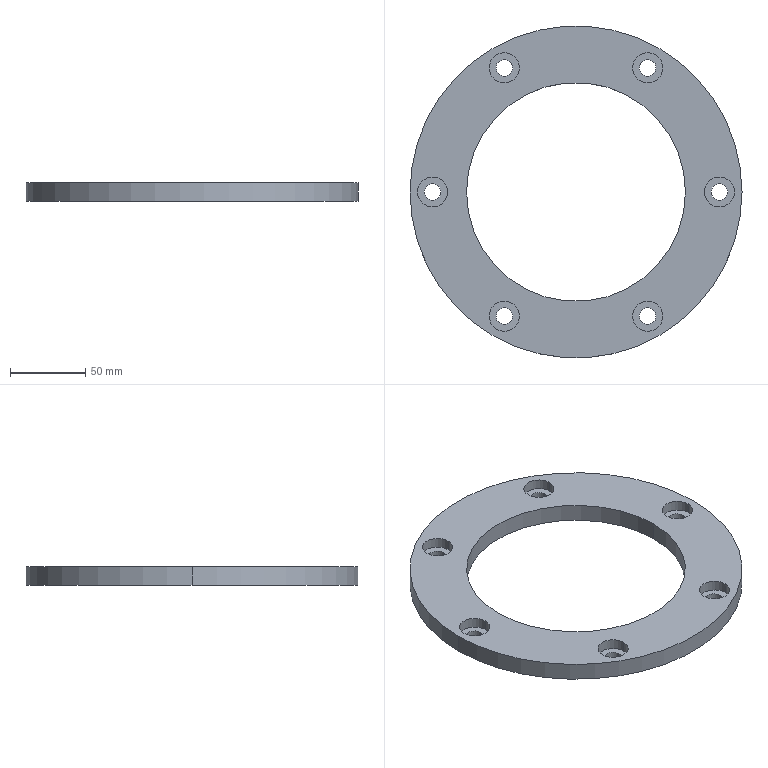Component | SolidWorks | PunchRetainer-1 | 1 solid | 36 faces | box 220 x 220 x 12 mm | volume 241958 mm3 | cylinder 28 | plane 8 | commonest cylinder face diameters 20 x12 11 x12 145 x2 220 x2
build123d program:
from build123d import *

# Parameters (mm, degrees)
SKETCH1_R           = 110
SKETCH1_R_2         = 72.5
SKETCH1_R_3         = 5.5
BOSS_EXTRUDE1_DEPTH = 12
SKETCH2_R           = 10
CUT_EXTRUDE1_DEPTH  = 7


with BuildPart() as part:
    # Sketch1 → Boss-Extrude1 (new body)
    with BuildSketch(Plane.XY):
        Circle(SKETCH1_R)
        Circle(SKETCH1_R_2, mode=Mode.SUBTRACT)
        with Locations((-95, 0)):
            Circle(SKETCH1_R_3, mode=Mode.SUBTRACT)
        with Locations((-47.5, 82.272)):
            Circle(SKETCH1_R_3, mode=Mode.SUBTRACT)
        with Locations((47.5, 82.272)):
            Circle(SKETCH1_R_3, mode=Mode.SUBTRACT)
        with Locations((95, 0)):
            Circle(SKETCH1_R_3, mode=Mode.SUBTRACT)
        with Locations((47.5, -82.272)):
            Circle(SKETCH1_R_3, mode=Mode.SUBTRACT)
        with Locations((-47.5, -82.272)):
            Circle(SKETCH1_R_3, mode=Mode.SUBTRACT)
    extrude(amount=BOSS_EXTRUDE1_DEPTH)

    # Sketch2 → Cut-Extrude1 (cut)
    with BuildSketch(Plane.XY.offset(12)):
        with Locations((-95, 0)):
            Circle(SKETCH2_R)
        with Locations((-47.5, 82.272)):
            Circle(SKETCH2_R)
        with Locations((47.5, 82.272)):
            Circle(SKETCH2_R)
        with Locations((95, 0)):
            Circle(SKETCH2_R)
        with Locations((47.5, -82.272)):
            Circle(SKETCH2_R)
        with Locations((-47.5, -82.272)):
            Circle(SKETCH2_R)
    extrude(amount=-CUT_EXTRUDE1_DEPTH, mode=Mode.SUBTRACT)


solid = part.part

# Placed as in the assembly
solid = solid.moved(Location((0, 0, -231), (0, 0, 0)))
STEP:
#1=COLOUR_RGB('',0.7922,0.8196,0.9333);
#2=FILL_AREA_STYLE_COLOUR('',#1);
#3=FILL_AREA_STYLE('',(#2));
#4=SURFACE_STYLE_FILL_AREA(#3);
#5=SURFACE_SIDE_STYLE('',(#4));
#6=SURFACE_STYLE_USAGE(.BOTH.,#5);
#7=PRESENTATION_STYLE_ASSIGNMENT((#6));
#8=CARTESIAN_POINT('',(-4.134,-0.,-8.898));
#9=VERTEX_POINT('',#8);
#10=CARTESIAN_POINT('',(-3.346,-0.,-8.898));
#11=VERTEX_POINT('',#10);
#12=CARTESIAN_POINT('',(-3.74,-0.,-8.898));
#13=DIRECTION('',(0.,0.,1.));
#14=DIRECTION('',(1.,0.,0.));
#15=AXIS2_PLACEMENT_3D('',#12,#13,#14);
#16=CIRCLE('',#15,0.3937);
#17=EDGE_CURVE('',#9,#11,#16,.T.);
#18=ORIENTED_EDGE('',*,*,#17,.F.);
#19=CARTESIAN_POINT('',(-4.134,-0.,-8.622));
#20=VERTEX_POINT('',#19);
#21=CARTESIAN_POINT('',(-4.134,-0.,-8.898));
#22=DIRECTION('',(0.,0.,1.));
#23=VECTOR('',#22,39.37);
#24=LINE('',#21,#23);
#25=EDGE_CURVE('',#9,#20,#24,.T.);
#26=ORIENTED_EDGE('',*,*,#25,.T.);
#27=CARTESIAN_POINT('',(-3.346,-0.,-8.622));
#28=VERTEX_POINT('',#27);
#29=CARTESIAN_POINT('',(-3.74,-0.,-8.622));
#30=DIRECTION('',(0.,0.,1.));
#31=DIRECTION('',(1.,0.,0.));
#32=AXIS2_PLACEMENT_3D('',#29,#30,#31);
#33=CIRCLE('',#32,0.3937);
#34=EDGE_CURVE('',#20,#28,#33,.T.);
#35=ORIENTED_EDGE('',*,*,#34,.T.);
#36=CARTESIAN_POINT('',(-3.346,-0.,-8.898));
#37=DIRECTION('',(0.,0.,1.));
#38=VECTOR('',#37,39.37);
#39=LINE('',#36,#38);
#40=EDGE_CURVE('',#11,#28,#39,.T.);
#41=ORIENTED_EDGE('',*,*,#40,.F.);
#42=EDGE_LOOP('',(#18,#26,#35,#41));
#43=FACE_OUTER_BOUND('',#42,.T.);
#44=CARTESIAN_POINT('',(-3.74,-0.,-8.898));
#45=DIRECTION('',(0.,0.,1.));
#46=DIRECTION('',(1.,0.,0.));
#47=AXIS2_PLACEMENT_3D('',#44,#45,#46);
#48=CYLINDRICAL_SURFACE('',#47,0.3937);
#49=ADVANCED_FACE('',(#43),#48,.F.);
#50=CARTESIAN_POINT('',(-2.264,3.239,-8.898));
#51=VERTEX_POINT('',#50);
#52=CARTESIAN_POINT('',(-1.476,3.239,-8.898));
#53=VERTEX_POINT('',#52);
#54=CARTESIAN_POINT('',(-1.87,3.239,-8.898));
#55=DIRECTION('',(0.,0.,1.));
#56=DIRECTION('',(1.,0.,0.));
#57=AXIS2_PLACEMENT_3D('',#54,#55,#56);
#58=CIRCLE('',#57,0.3937);
#59=EDGE_CURVE('',#51,#53,#58,.T.);
#60=ORIENTED_EDGE('',*,*,#59,.F.);
#61=CARTESIAN_POINT('',(-2.264,3.239,-8.622));
#62=VERTEX_POINT('',#61);
#63=CARTESIAN_POINT('',(-2.264,3.239,-8.898));
#64=DIRECTION('',(0.,0.,1.));
#65=VECTOR('',#64,39.37);
#66=LINE('',#63,#65);
#67=EDGE_CURVE('',#51,#62,#66,.T.);
#68=ORIENTED_EDGE('',*,*,#67,.T.);
#69=CARTESIAN_POINT('',(-1.476,3.239,-8.622));
#70=VERTEX_POINT('',#69);
#71=CARTESIAN_POINT('',(-1.87,3.239,-8.622));
#72=DIRECTION('',(0.,0.,1.));
#73=DIRECTION('',(1.,0.,0.));
#74=AXIS2_PLACEMENT_3D('',#71,#72,#73);
#75=CIRCLE('',#74,0.3937);
#76=EDGE_CURVE('',#62,#70,#75,.T.);
#77=ORIENTED_EDGE('',*,*,#76,.T.);
#78=CARTESIAN_POINT('',(-1.476,3.239,-8.898));
#79=DIRECTION('',(0.,0.,1.));
#80=VECTOR('',#79,39.37);
#81=LINE('',#78,#80);
#82=EDGE_CURVE('',#53,#70,#81,.T.);
#83=ORIENTED_EDGE('',*,*,#82,.F.);
#84=EDGE_LOOP('',(#60,#68,#77,#83));
#85=FACE_OUTER_BOUND('',#84,.T.);
#86=CARTESIAN_POINT('',(-1.87,3.239,-8.898));
#87=DIRECTION('',(0.,0.,1.));
#88=DIRECTION('',(1.,0.,0.));
#89=AXIS2_PLACEMENT_3D('',#86,#87,#88);
#90=CYLINDRICAL_SURFACE('',#89,0.3937);
#91=ADVANCED_FACE('',(#85),#90,.F.);
#92=CARTESIAN_POINT('',(1.476,3.239,-8.898));
#93=VERTEX_POINT('',#92);
#94=CARTESIAN_POINT('',(2.264,3.239,-8.898));
#95=VERTEX_POINT('',#94);
#96=CARTESIAN_POINT('',(1.87,3.239,-8.898));
#97=DIRECTION('',(0.,0.,1.));
#98=DIRECTION('',(1.,0.,0.));
#99=AXIS2_PLACEMENT_3D('',#96,#97,#98);
#100=CIRCLE('',#99,0.3937);
#101=EDGE_CURVE('',#93,#95,#100,.T.);
#102=ORIENTED_EDGE('',*,*,#101,.F.);
#103=CARTESIAN_POINT('',(1.476,3.239,-8.622));
#104=VERTEX_POINT('',#103);
#105=CARTESIAN_POINT('',(1.476,3.239,-8.898));
#106=DIRECTION('',(0.,0.,1.));
#107=VECTOR('',#106,39.37);
#108=LINE('',#105,#107);
#109=EDGE_CURVE('',#93,#104,#108,.T.);
#110=ORIENTED_EDGE('',*,*,#109,.T.);
#111=CARTESIAN_POINT('',(2.264,3.239,-8.622));
#112=VERTEX_POINT('',#111);
#113=CARTESIAN_POINT('',(1.87,3.239,-8.622));
#114=DIRECTION('',(0.,0.,1.));
#115=DIRECTION('',(1.,0.,0.));
#116=AXIS2_PLACEMENT_3D('',#113,#114,#115);
#117=CIRCLE('',#116,0.3937);
#118=EDGE_CURVE('',#104,#112,#117,.T.);
#119=ORIENTED_EDGE('',*,*,#118,.T.);
#120=CARTESIAN_POINT('',(2.264,3.239,-8.898));
#121=DIRECTION('',(0.,0.,1.));
#122=VECTOR('',#121,39.37);
#123=LINE('',#120,#122);
#124=EDGE_CURVE('',#95,#112,#123,.T.);
#125=ORIENTED_EDGE('',*,*,#124,.F.);
#126=EDGE_LOOP('',(#102,#110,#119,#125));
#127=FACE_OUTER_BOUND('',#126,.T.);
#128=CARTESIAN_POINT('',(1.87,3.239,-8.898));
#129=DIRECTION('',(0.,0.,1.));
#130=DIRECTION('',(1.,0.,0.));
#131=AXIS2_PLACEMENT_3D('',#128,#129,#130);
#132=CYLINDRICAL_SURFACE('',#131,0.3937);
#133=ADVANCED_FACE('',(#127),#132,.F.);
#134=CARTESIAN_POINT('',(3.346,0.,-8.898));
#135=VERTEX_POINT('',#134);
#136=CARTESIAN_POINT('',(4.134,0.,-8.898));
#137=VERTEX_POINT('',#136);
#138=CARTESIAN_POINT('',(3.74,0.,-8.898));
#139=DIRECTION('',(0.,0.,1.));
#140=DIRECTION('',(1.,0.,0.));
#141=AXIS2_PLACEMENT_3D('',#138,#139,#140);
#142=CIRCLE('',#141,0.3937);
#143=EDGE_CURVE('',#135,#137,#142,.T.);
#144=ORIENTED_EDGE('',*,*,#143,.F.);
#145=CARTESIAN_POINT('',(3.346,0.,-8.622));
#146=VERTEX_POINT('',#145);
#147=CARTESIAN_POINT('',(3.346,0.,-8.898));
#148=DIRECTION('',(0.,0.,1.));
#149=VECTOR('',#148,39.37);
#150=LINE('',#147,#149);
#151=EDGE_CURVE('',#135,#146,#150,.T.);
#152=ORIENTED_EDGE('',*,*,#151,.T.);
#153=CARTESIAN_POINT('',(4.134,0.,-8.622));
#154=VERTEX_POINT('',#153);
#155=CARTESIAN_POINT('',(3.74,0.,-8.622));
#156=DIRECTION('',(0.,0.,1.));
#157=DIRECTION('',(1.,0.,0.));
#158=AXIS2_PLACEMENT_3D('',#155,#156,#157);
#159=CIRCLE('',#158,0.3937);
#160=EDGE_CURVE('',#146,#154,#159,.T.);
#161=ORIENTED_EDGE('',*,*,#160,.T.);
#162=CARTESIAN_POINT('',(4.134,0.,-8.898));
#163=DIRECTION('',(0.,0.,1.));
#164=VECTOR('',#163,39.37);
#165=LINE('',#162,#164);
#166=EDGE_CURVE('',#137,#154,#165,.T.);
#167=ORIENTED_EDGE('',*,*,#166,.F.);
#168=EDGE_LOOP('',(#144,#152,#161,#167));
#169=FACE_OUTER_BOUND('',#168,.T.);
#170=CARTESIAN_POINT('',(3.74,0.,-8.898));
#171=DIRECTION('',(0.,0.,1.));
#172=DIRECTION('',(1.,0.,0.));
#173=AXIS2_PLACEMENT_3D('',#170,#171,#172);
#174=CYLINDRICAL_SURFACE('',#173,0.3937);
#175=ADVANCED_FACE('',(#169),#174,.F.);
#176=CARTESIAN_POINT('',(1.476,-3.239,-8.898));
#177=VERTEX_POINT('',#176);
#178=CARTESIAN_POINT('',(2.264,-3.239,-8.898));
#179=VERTEX_POINT('',#178);
#180=CARTESIAN_POINT('',(1.87,-3.239,-8.898));
#181=DIRECTION('',(0.,0.,1.));
#182=DIRECTION('',(1.,0.,0.));
#183=AXIS2_PLACEMENT_3D('',#180,#181,#182);
#184=CIRCLE('',#183,0.3937);
#185=EDGE_CURVE('',#177,#179,#184,.T.);
#186=ORIENTED_EDGE('',*,*,#185,.F.);
#187=CARTESIAN_POINT('',(1.476,-3.239,-8.622));
#188=VERTEX_POINT('',#187);
#189=CARTESIAN_POINT('',(1.476,-3.239,-8.898));
#190=DIRECTION('',(0.,0.,1.));
#191=VECTOR('',#190,39.37);
#192=LINE('',#189,#191);
#193=EDGE_CURVE('',#177,#188,#192,.T.);
#194=ORIENTED_EDGE('',*,*,#193,.T.);
#195=CARTESIAN_POINT('',(2.264,-3.239,-8.622));
#196=VERTEX_POINT('',#195);
#197=CARTESIAN_POINT('',(1.87,-3.239,-8.622));
#198=DIRECTION('',(0.,0.,1.));
#199=DIRECTION('',(1.,0.,0.));
#200=AXIS2_PLACEMENT_3D('',#197,#198,#199);
#201=CIRCLE('',#200,0.3937);
#202=EDGE_CURVE('',#188,#196,#201,.T.);
#203=ORIENTED_EDGE('',*,*,#202,.T.);
#204=CARTESIAN_POINT('',(2.264,-3.239,-8.898));
#205=DIRECTION('',(0.,0.,1.));
#206=VECTOR('',#205,39.37);
#207=LINE('',#204,#206);
#208=EDGE_CURVE('',#179,#196,#207,.T.);
#209=ORIENTED_EDGE('',*,*,#208,.F.);
#210=EDGE_LOOP('',(#186,#194,#203,#209));
#211=FACE_OUTER_BOUND('',#210,.T.);
#212=CARTESIAN_POINT('',(1.87,-3.239,-8.898));
#213=DIRECTION('',(0.,0.,1.));
#214=DIRECTION('',(1.,0.,0.));
#215=AXIS2_PLACEMENT_3D('',#212,#213,#214);
#216=CYLINDRICAL_SURFACE('',#215,0.3937);
#217=ADVANCED_FACE('',(#211),#216,.F.);
#218=CARTESIAN_POINT('',(-2.264,-3.239,-8.898));
#219=VERTEX_POINT('',#218);
#220=CARTESIAN_POINT('',(-1.476,-3.239,-8.898));
#221=VERTEX_POINT('',#220);
#222=CARTESIAN_POINT('',(-1.87,-3.239,-8.898));
#223=DIRECTION('',(0.,0.,1.));
#224=DIRECTION('',(1.,0.,0.));
#225=AXIS2_PLACEMENT_3D('',#222,#223,#224);
#226=CIRCLE('',#225,0.3937);
#227=EDGE_CURVE('',#219,#221,#226,.T.);
#228=ORIENTED_EDGE('',*,*,#227,.F.);
#229=CARTESIAN_POINT('',(-2.264,-3.239,-8.622));
#230=VERTEX_POINT('',#229);
#231=CARTESIAN_POINT('',(-2.264,-3.239,-8.898));
#232=DIRECTION('',(0.,0.,1.));
#233=VECTOR('',#232,39.37);
#234=LINE('',#231,#233);
#235=EDGE_CURVE('',#219,#230,#234,.T.);
#236=ORIENTED_EDGE('',*,*,#235,.T.);
#237=CARTESIAN_POINT('',(-1.476,-3.239,-8.622));
#238=VERTEX_POINT('',#237);
#239=CARTESIAN_POINT('',(-1.87,-3.239,-8.622));
#240=DIRECTION('',(0.,0.,1.));
#241=DIRECTION('',(1.,0.,0.));
#242=AXIS2_PLACEMENT_3D('',#239,#240,#241);
#243=CIRCLE('',#242,0.3937);
#244=EDGE_CURVE('',#230,#238,#243,.T.);
#245=ORIENTED_EDGE('',*,*,#244,.T.);
#246=CARTESIAN_POINT('',(-1.476,-3.239,-8.898));
#247=DIRECTION('',(0.,0.,1.));
#248=VECTOR('',#247,39.37);
#249=LINE('',#246,#248);
#250=EDGE_CURVE('',#221,#238,#249,.T.);
#251=ORIENTED_EDGE('',*,*,#250,.F.);
#252=EDGE_LOOP('',(#228,#236,#245,#251));
#253=FACE_OUTER_BOUND('',#252,.T.);
#254=CARTESIAN_POINT('',(-1.87,-3.239,-8.898));
#255=DIRECTION('',(0.,0.,1.));
#256=DIRECTION('',(1.,0.,0.));
#257=AXIS2_PLACEMENT_3D('',#254,#255,#256);
#258=CYLINDRICAL_SURFACE('',#257,0.3937);
#259=ADVANCED_FACE('',(#253),#258,.F.);
#260=CARTESIAN_POINT('',(-2.854,-0.,-8.622));
#261=VERTEX_POINT('',#260);
#262=CARTESIAN_POINT('',(2.854,-0.,-8.622));
#263=VERTEX_POINT('',#262);
#264=CARTESIAN_POINT('',(-0.,-0.,-8.622));
#265=DIRECTION('',(0.,0.,1.));
#266=DIRECTION('',(1.,0.,0.));
#267=AXIS2_PLACEMENT_3D('',#264,#265,#266);
#268=CIRCLE('',#267,2.854);
#269=EDGE_CURVE('',#261,#263,#268,.T.);
#270=ORIENTED_EDGE('',*,*,#269,.T.);
#271=CARTESIAN_POINT('',(2.854,-0.,-9.094));
#272=VERTEX_POINT('',#271);
#273=CARTESIAN_POINT('',(2.854,-0.,-8.622));
#274=DIRECTION('',(0.,0.,-1.));
#275=VECTOR('',#274,39.37);
#276=LINE('',#273,#275);
#277=EDGE_CURVE('',#263,#272,#276,.T.);
#278=ORIENTED_EDGE('',*,*,#277,.T.);
#279=CARTESIAN_POINT('',(-2.854,-0.,-9.094));
#280=VERTEX_POINT('',#279);
#281=CARTESIAN_POINT('',(-0.,-0.,-9.094));
#282=DIRECTION('',(0.,0.,1.));
#283=DIRECTION('',(1.,0.,0.));
#284=AXIS2_PLACEMENT_3D('',#281,#282,#283);
#285=CIRCLE('',#284,2.854);
#286=EDGE_CURVE('',#280,#272,#285,.T.);
#287=ORIENTED_EDGE('',*,*,#286,.F.);
#288=CARTESIAN_POINT('',(-2.854,-0.,-8.622));
#289=DIRECTION('',(0.,0.,-1.));
#290=VECTOR('',#289,39.37);
#291=LINE('',#288,#290);
#292=EDGE_CURVE('',#261,#280,#291,.T.);
#293=ORIENTED_EDGE('',*,*,#292,.F.);
#294=EDGE_LOOP('',(#270,#278,#287,#293));
#295=FACE_OUTER_BOUND('',#294,.T.);
#296=CARTESIAN_POINT('',(-0.,-0.,-8.622));
#297=DIRECTION('',(0.,0.,-1.));
#298=DIRECTION('',(-1.,0.,0.));
#299=AXIS2_PLACEMENT_3D('',#296,#297,#298);
#300=CYLINDRICAL_SURFACE('',#299,2.854);
#301=ADVANCED_FACE('',(#295),#300,.F.);
#302=CARTESIAN_POINT('',(4.331,-0.,-8.622));
#303=VERTEX_POINT('',#302);
#304=CARTESIAN_POINT('',(-4.331,-0.,-8.622));
#305=VERTEX_POINT('',#304);
#306=CARTESIAN_POINT('',(-0.,-0.,-8.622));
#307=DIRECTION('',(0.,0.,1.));
#308=DIRECTION('',(1.,0.,0.));
#309=AXIS2_PLACEMENT_3D('',#306,#307,#308);
#310=CIRCLE('',#309,4.331);
#311=EDGE_CURVE('',#303,#305,#310,.T.);
#312=ORIENTED_EDGE('',*,*,#311,.F.);
#313=CARTESIAN_POINT('',(4.331,-0.,-9.094));
#314=VERTEX_POINT('',#313);
#315=CARTESIAN_POINT('',(4.331,-0.,-8.622));
#316=DIRECTION('',(0.,0.,-1.));
#317=VECTOR('',#316,39.37);
#318=LINE('',#315,#317);
#319=EDGE_CURVE('',#303,#314,#318,.T.);
#320=ORIENTED_EDGE('',*,*,#319,.T.);
#321=CARTESIAN_POINT('',(-4.331,-0.,-9.094));
#322=VERTEX_POINT('',#321);
#323=CARTESIAN_POINT('',(-0.,-0.,-9.094));
#324=DIRECTION('',(0.,0.,1.));
#325=DIRECTION('',(1.,0.,0.));
#326=AXIS2_PLACEMENT_3D('',#323,#324,#325);
#327=CIRCLE('',#326,4.331);
#328=EDGE_CURVE('',#314,#322,#327,.T.);
#329=ORIENTED_EDGE('',*,*,#328,.T.);
#330=CARTESIAN_POINT('',(-4.331,-0.,-8.622));
#331=DIRECTION('',(0.,0.,-1.));
#332=VECTOR('',#331,39.37);
#333=LINE('',#330,#332);
#334=EDGE_CURVE('',#305,#322,#333,.T.);
#335=ORIENTED_EDGE('',*,*,#334,.F.);
#336=EDGE_LOOP('',(#312,#320,#329,#335));
#337=FACE_OUTER_BOUND('',#336,.T.);
#338=CARTESIAN_POINT('',(-0.,-0.,-8.622));
#339=DIRECTION('',(0.,0.,-1.));
#340=DIRECTION('',(-1.,0.,0.));
#341=AXIS2_PLACEMENT_3D('',#338,#339,#340);
#342=CYLINDRICAL_SURFACE('',#341,4.331);
#343=ADVANCED_FACE('',(#337),#342,.T.);
#344=CARTESIAN_POINT('',(-2.087,-3.239,-8.898));
#345=VERTEX_POINT('',#344);
#346=CARTESIAN_POINT('',(-1.654,-3.239,-8.898));
#347=VERTEX_POINT('',#346);
#348=CARTESIAN_POINT('',(-1.87,-3.239,-8.898));
#349=DIRECTION('',(0.,0.,1.));
#350=DIRECTION('',(1.,0.,0.));
#351=AXIS2_PLACEMENT_3D('',#348,#349,#350);
#352=CIRCLE('',#351,0.2165);
#353=EDGE_CURVE('',#345,#347,#352,.T.);
#354=ORIENTED_EDGE('',*,*,#353,.T.);
#355=CARTESIAN_POINT('',(-1.654,-3.239,-9.094));
#356=VERTEX_POINT('',#355);
#357=CARTESIAN_POINT('',(-1.654,-3.239,-8.622));
#358=DIRECTION('',(0.,0.,-1.));
#359=VECTOR('',#358,39.37);
#360=LINE('',#357,#359);
#361=EDGE_CURVE('',#347,#356,#360,.T.);
#362=ORIENTED_EDGE('',*,*,#361,.T.);
#363=CARTESIAN_POINT('',(-2.087,-3.239,-9.094));
#364=VERTEX_POINT('',#363);
#365=CARTESIAN_POINT('',(-1.87,-3.239,-9.094));
#366=DIRECTION('',(0.,0.,1.));
#367=DIRECTION('',(1.,0.,0.));
#368=AXIS2_PLACEMENT_3D('',#365,#366,#367);
#369=CIRCLE('',#368,0.2165);
#370=EDGE_CURVE('',#364,#356,#369,.T.);
#371=ORIENTED_EDGE('',*,*,#370,.F.);
#372=CARTESIAN_POINT('',(-2.087,-3.239,-8.622));
#373=DIRECTION('',(0.,0.,-1.));
#374=VECTOR('',#373,39.37);
#375=LINE('',#372,#374);
#376=EDGE_CURVE('',#345,#364,#375,.T.);
#377=ORIENTED_EDGE('',*,*,#376,.F.);
#378=EDGE_LOOP('',(#354,#362,#371,#377));
#379=FACE_OUTER_BOUND('',#378,.T.);
#380=CARTESIAN_POINT('',(-1.87,-3.239,-8.622));
#381=DIRECTION('',(0.,0.,-1.));
#382=DIRECTION('',(-1.,0.,0.));
#383=AXIS2_PLACEMENT_3D('',#380,#381,#382);
#384=CYLINDRICAL_SURFACE('',#383,0.2165);
#385=ADVANCED_FACE('',(#379),#384,.F.);
#386=CARTESIAN_POINT('',(1.654,-3.239,-8.898));
#387=VERTEX_POINT('',#386);
#388=CARTESIAN_POINT('',(2.087,-3.239,-8.898));
#389=VERTEX_POINT('',#388);
#390=CARTESIAN_POINT('',(1.87,-3.239,-8.898));
#391=DIRECTION('',(0.,0.,1.));
#392=DIRECTION('',(1.,0.,0.));
#393=AXIS2_PLACEMENT_3D('',#390,#391,#392);
#394=CIRCLE('',#393,0.2165);
#395=EDGE_CURVE('',#387,#389,#394,.T.);
#396=ORIENTED_EDGE('',*,*,#395,.T.);
#397=CARTESIAN_POINT('',(2.087,-3.239,-9.094));
#398=VERTEX_POINT('',#397);
#399=CARTESIAN_POINT('',(2.087,-3.239,-8.622));
#400=DIRECTION('',(0.,0.,-1.));
#401=VECTOR('',#400,39.37);
#402=LINE('',#399,#401);
#403=EDGE_CURVE('',#389,#398,#402,.T.);
#404=ORIENTED_EDGE('',*,*,#403,.T.);
#405=CARTESIAN_POINT('',(1.654,-3.239,-9.094));
#406=VERTEX_POINT('',#405);
#407=CARTESIAN_POINT('',(1.87,-3.239,-9.094));
#408=DIRECTION('',(0.,0.,1.));
#409=DIRECTION('',(1.,0.,0.));
#410=AXIS2_PLACEMENT_3D('',#407,#408,#409);
#411=CIRCLE('',#410,0.2165);
#412=EDGE_CURVE('',#406,#398,#411,.T.);
#413=ORIENTED_EDGE('',*,*,#412,.F.);
#414=CARTESIAN_POINT('',(1.654,-3.239,-8.622));
#415=DIRECTION('',(0.,0.,-1.));
#416=VECTOR('',#415,39.37);
#417=LINE('',#414,#416);
#418=EDGE_CURVE('',#387,#406,#417,.T.);
#419=ORIENTED_EDGE('',*,*,#418,.F.);
#420=EDGE_LOOP('',(#396,#404,#413,#419));
#421=FACE_OUTER_BOUND('',#420,.T.);
#422=CARTESIAN_POINT('',(1.87,-3.239,-8.622));
#423=DIRECTION('',(0.,0.,-1.));
#424=DIRECTION('',(-1.,0.,0.));
#425=AXIS2_PLACEMENT_3D('',#422,#423,#424);
#426=CYLINDRICAL_SURFACE('',#425,0.2165);
#427=ADVANCED_FACE('',(#421),#426,.F.);
#428=CARTESIAN_POINT('',(3.524,-0.,-8.898));
#429=VERTEX_POINT('',#428);
#430=CARTESIAN_POINT('',(3.957,-0.,-8.898));
#431=VERTEX_POINT('',#430);
#432=CARTESIAN_POINT('',(3.74,-0.,-8.898));
#433=DIRECTION('',(0.,0.,1.));
#434=DIRECTION('',(1.,0.,0.));
#435=AXIS2_PLACEMENT_3D('',#432,#433,#434);
#436=CIRCLE('',#435,0.2165);
#437=EDGE_CURVE('',#429,#431,#436,.T.);
#438=ORIENTED_EDGE('',*,*,#437,.T.);
#439=CARTESIAN_POINT('',(3.957,-0.,-9.094));
#440=VERTEX_POINT('',#439);
#441=CARTESIAN_POINT('',(3.957,-0.,-8.622));
#442=DIRECTION('',(0.,0.,-1.));
#443=VECTOR('',#442,39.37);
#444=LINE('',#441,#443);
#445=EDGE_CURVE('',#431,#440,#444,.T.);
#446=ORIENTED_EDGE('',*,*,#445,.T.);
#447=CARTESIAN_POINT('',(3.524,-0.,-9.094));
#448=VERTEX_POINT('',#447);
#449=CARTESIAN_POINT('',(3.74,-0.,-9.094));
#450=DIRECTION('',(0.,0.,1.));
#451=DIRECTION('',(1.,0.,0.));
#452=AXIS2_PLACEMENT_3D('',#449,#450,#451);
#453=CIRCLE('',#452,0.2165);
#454=EDGE_CURVE('',#448,#440,#453,.T.);
#455=ORIENTED_EDGE('',*,*,#454,.F.);
#456=CARTESIAN_POINT('',(3.524,-0.,-8.622));
#457=DIRECTION('',(0.,0.,-1.));
#458=VECTOR('',#457,39.37);
#459=LINE('',#456,#458);
#460=EDGE_CURVE('',#429,#448,#459,.T.);
#461=ORIENTED_EDGE('',*,*,#460,.F.);
#462=EDGE_LOOP('',(#438,#446,#455,#461));
#463=FACE_OUTER_BOUND('',#462,.T.);
#464=CARTESIAN_POINT('',(3.74,-0.,-8.622));
#465=DIRECTION('',(0.,0.,-1.));
#466=DIRECTION('',(-1.,0.,0.));
#467=AXIS2_PLACEMENT_3D('',#464,#465,#466);
#468=CYLINDRICAL_SURFACE('',#467,0.2165);
#469=ADVANCED_FACE('',(#463),#468,.F.);
#470=CARTESIAN_POINT('',(1.654,3.239,-8.898));
#471=VERTEX_POINT('',#470);
#472=CARTESIAN_POINT('',(2.087,3.239,-8.898));
#473=VERTEX_POINT('',#472);
#474=CARTESIAN_POINT('',(1.87,3.239,-8.898));
#475=DIRECTION('',(0.,0.,1.));
#476=DIRECTION('',(1.,0.,0.));
#477=AXIS2_PLACEMENT_3D('',#474,#475,#476);
#478=CIRCLE('',#477,0.2165);
#479=EDGE_CURVE('',#471,#473,#478,.T.);
#480=ORIENTED_EDGE('',*,*,#479,.T.);
#481=CARTESIAN_POINT('',(2.087,3.239,-9.094));
#482=VERTEX_POINT('',#481);
#483=CARTESIAN_POINT('',(2.087,3.239,-8.622));
#484=DIRECTION('',(0.,0.,-1.));
#485=VECTOR('',#484,39.37);
#486=LINE('',#483,#485);
#487=EDGE_CURVE('',#473,#482,#486,.T.);
#488=ORIENTED_EDGE('',*,*,#487,.T.);
#489=CARTESIAN_POINT('',(1.654,3.239,-9.094));
#490=VERTEX_POINT('',#489);
#491=CARTESIAN_POINT('',(1.87,3.239,-9.094));
#492=DIRECTION('',(0.,0.,1.));
#493=DIRECTION('',(1.,0.,0.));
#494=AXIS2_PLACEMENT_3D('',#491,#492,#493);
#495=CIRCLE('',#494,0.2165);
#496=EDGE_CURVE('',#490,#482,#495,.T.);
#497=ORIENTED_EDGE('',*,*,#496,.F.);
#498=CARTESIAN_POINT('',(1.654,3.239,-8.622));
#499=DIRECTION('',(0.,0.,-1.));
#500=VECTOR('',#499,39.37);
#501=LINE('',#498,#500);
#502=EDGE_CURVE('',#471,#490,#501,.T.);
#503=ORIENTED_EDGE('',*,*,#502,.F.);
#504=EDGE_LOOP('',(#480,#488,#497,#503));
#505=FACE_OUTER_BOUND('',#504,.T.);
#506=CARTESIAN_POINT('',(1.87,3.239,-8.622));
#507=DIRECTION('',(0.,0.,-1.));
#508=DIRECTION('',(-1.,0.,0.));
#509=AXIS2_PLACEMENT_3D('',#506,#507,#508);
#510=CYLINDRICAL_SURFACE('',#509,0.2165);
#511=ADVANCED_FACE('',(#505),#510,.F.);
#512=CARTESIAN_POINT('',(-2.087,3.239,-8.898));
#513=VERTEX_POINT('',#512);
#514=CARTESIAN_POINT('',(-1.654,3.239,-8.898));
#515=VERTEX_POINT('',#514);
#516=CARTESIAN_POINT('',(-1.87,3.239,-8.898));
#517=DIRECTION('',(0.,0.,1.));
#518=DIRECTION('',(1.,0.,0.));
#519=AXIS2_PLACEMENT_3D('',#516,#517,#518);
#520=CIRCLE('',#519,0.2165);
#521=EDGE_CURVE('',#513,#515,#520,.T.);
#522=ORIENTED_EDGE('',*,*,#521,.T.);
#523=CARTESIAN_POINT('',(-1.654,3.239,-9.094));
#524=VERTEX_POINT('',#523);
#525=CARTESIAN_POINT('',(-1.654,3.239,-8.622));
#526=DIRECTION('',(0.,0.,-1.));
#527=VECTOR('',#526,39.37);
#528=LINE('',#525,#527);
#529=EDGE_CURVE('',#515,#524,#528,.T.);
#530=ORIENTED_EDGE('',*,*,#529,.T.);
#531=CARTESIAN_POINT('',(-2.087,3.239,-9.094));
#532=VERTEX_POINT('',#531);
#533=CARTESIAN_POINT('',(-1.87,3.239,-9.094));
#534=DIRECTION('',(0.,0.,1.));
#535=DIRECTION('',(1.,0.,0.));
#536=AXIS2_PLACEMENT_3D('',#533,#534,#535);
#537=CIRCLE('',#536,0.2165);
#538=EDGE_CURVE('',#532,#524,#537,.T.);
#539=ORIENTED_EDGE('',*,*,#538,.F.);
#540=CARTESIAN_POINT('',(-2.087,3.239,-8.622));
#541=DIRECTION('',(0.,0.,-1.));
#542=VECTOR('',#541,39.37);
#543=LINE('',#540,#542);
#544=EDGE_CURVE('',#513,#532,#543,.T.);
#545=ORIENTED_EDGE('',*,*,#544,.F.);
#546=EDGE_LOOP('',(#522,#530,#539,#545));
#547=FACE_OUTER_BOUND('',#546,.T.);
#548=CARTESIAN_POINT('',(-1.87,3.239,-8.622));
#549=DIRECTION('',(0.,0.,-1.));
#550=DIRECTION('',(-1.,0.,0.));
#551=AXIS2_PLACEMENT_3D('',#548,#549,#550);
#552=CYLINDRICAL_SURFACE('',#551,0.2165);
#553=ADVANCED_FACE('',(#547),#552,.F.);
#554=CARTESIAN_POINT('',(-3.957,-0.,-8.898));
#555=VERTEX_POINT('',#554);
#556=CARTESIAN_POINT('',(-3.524,-0.,-8.898));
#557=VERTEX_POINT('',#556);
#558=CARTESIAN_POINT('',(-3.74,-0.,-8.898));
#559=DIRECTION('',(0.,0.,1.));
#560=DIRECTION('',(1.,0.,0.));
#561=AXIS2_PLACEMENT_3D('',#558,#559,#560);
#562=CIRCLE('',#561,0.2165);
#563=EDGE_CURVE('',#555,#557,#562,.T.);
#564=ORIENTED_EDGE('',*,*,#563,.T.);
#565=CARTESIAN_POINT('',(-3.524,-0.,-9.094));
#566=VERTEX_POINT('',#565);
#567=CARTESIAN_POINT('',(-3.524,-0.,-8.622));
#568=DIRECTION('',(0.,0.,-1.));
#569=VECTOR('',#568,39.37);
#570=LINE('',#567,#569);
#571=EDGE_CURVE('',#557,#566,#570,.T.);
#572=ORIENTED_EDGE('',*,*,#571,.T.);
#573=CARTESIAN_POINT('',(-3.957,-0.,-9.094));
#574=VERTEX_POINT('',#573);
#575=CARTESIAN_POINT('',(-3.74,-0.,-9.094));
#576=DIRECTION('',(0.,0.,1.));
#577=DIRECTION('',(1.,0.,0.));
#578=AXIS2_PLACEMENT_3D('',#575,#576,#577);
#579=CIRCLE('',#578,0.2165);
#580=EDGE_CURVE('',#574,#566,#579,.T.);
#581=ORIENTED_EDGE('',*,*,#580,.F.);
#582=CARTESIAN_POINT('',(-3.957,-0.,-8.622));
#583=DIRECTION('',(0.,0.,-1.));
#584=VECTOR('',#583,39.37);
#585=LINE('',#582,#584);
#586=EDGE_CURVE('',#555,#574,#585,.T.);
#587=ORIENTED_EDGE('',*,*,#586,.F.);
#588=EDGE_LOOP('',(#564,#572,#581,#587));
#589=FACE_OUTER_BOUND('',#588,.T.);
#590=CARTESIAN_POINT('',(-3.74,-0.,-8.622));
#591=DIRECTION('',(0.,0.,-1.));
#592=DIRECTION('',(-1.,0.,0.));
#593=AXIS2_PLACEMENT_3D('',#590,#591,#592);
#594=CYLINDRICAL_SURFACE('',#593,0.2165);
#595=ADVANCED_FACE('',(#589),#594,.F.);
#596=ORIENTED_EDGE('',*,*,#571,.F.);
#597=CARTESIAN_POINT('',(-3.74,-0.,-8.898));
#598=DIRECTION('',(0.,0.,1.));
#599=DIRECTION('',(1.,0.,0.));
#600=AXIS2_PLACEMENT_3D('',#597,#598,#599);
#601=CIRCLE('',#600,0.2165);
#602=EDGE_CURVE('',#557,#555,#601,.T.);
#603=ORIENTED_EDGE('',*,*,#602,.T.);
#604=ORIENTED_EDGE('',*,*,#586,.T.);
#605=CARTESIAN_POINT('',(-3.74,-0.,-9.094));
#606=DIRECTION('',(0.,0.,1.));
#607=DIRECTION('',(1.,0.,0.));
#608=AXIS2_PLACEMENT_3D('',#605,#606,#607);
#609=CIRCLE('',#608,0.2165);
#610=EDGE_CURVE('',#566,#574,#609,.T.);
#611=ORIENTED_EDGE('',*,*,#610,.F.);
#612=EDGE_LOOP('',(#596,#603,#604,#611));
#613=FACE_OUTER_BOUND('',#612,.T.);
#614=CARTESIAN_POINT('',(-3.74,-0.,-8.622));
#615=DIRECTION('',(0.,0.,-1.));
#616=DIRECTION('',(-1.,0.,0.));
#617=AXIS2_PLACEMENT_3D('',#614,#615,#616);
#618=CYLINDRICAL_SURFACE('',#617,0.2165);
#619=ADVANCED_FACE('',(#613),#618,.F.);
#620=ORIENTED_EDGE('',*,*,#529,.F.);
#621=CARTESIAN_POINT('',(-1.87,3.239,-8.898));
#622=DIRECTION('',(0.,0.,1.));
#623=DIRECTION('',(1.,0.,0.));
#624=AXIS2_PLACEMENT_3D('',#621,#622,#623);
#625=CIRCLE('',#624,0.2165);
#626=EDGE_CURVE('',#515,#513,#625,.T.);
#627=ORIENTED_EDGE('',*,*,#626,.T.);
#628=ORIENTED_EDGE('',*,*,#544,.T.);
#629=CARTESIAN_POINT('',(-1.87,3.239,-9.094));
#630=DIRECTION('',(0.,0.,1.));
#631=DIRECTION('',(1.,0.,0.));
#632=AXIS2_PLACEMENT_3D('',#629,#630,#631);
#633=CIRCLE('',#632,0.2165);
#634=EDGE_CURVE('',#524,#532,#633,.T.);
#635=ORIENTED_EDGE('',*,*,#634,.F.);
#636=EDGE_LOOP('',(#620,#627,#628,#635));
#637=FACE_OUTER_BOUND('',#636,.T.);
#638=CARTESIAN_POINT('',(-1.87,3.239,-8.622));
#639=DIRECTION('',(0.,0.,-1.));
#640=DIRECTION('',(-1.,0.,0.));
#641=AXIS2_PLACEMENT_3D('',#638,#639,#640);
#642=CYLINDRICAL_SURFACE('',#641,0.2165);
#643=ADVANCED_FACE('',(#637),#642,.F.);
#644=ORIENTED_EDGE('',*,*,#487,.F.);
#645=CARTESIAN_POINT('',(1.87,3.239,-8.898));
#646=DIRECTION('',(0.,0.,1.));
#647=DIRECTION('',(1.,0.,0.));
#648=AXIS2_PLACEMENT_3D('',#645,#646,#647);
#649=CIRCLE('',#648,0.2165);
#650=EDGE_CURVE('',#473,#471,#649,.T.);
#651=ORIENTED_EDGE('',*,*,#650,.T.);
#652=ORIENTED_EDGE('',*,*,#502,.T.);
#653=CARTESIAN_POINT('',(1.87,3.239,-9.094));
#654=DIRECTION('',(0.,0.,1.));
#655=DIRECTION('',(1.,0.,0.));
#656=AXIS2_PLACEMENT_3D('',#653,#654,#655);
#657=CIRCLE('',#656,0.2165);
#658=EDGE_CURVE('',#482,#490,#657,.T.);
#659=ORIENTED_EDGE('',*,*,#658,.F.);
#660=EDGE_LOOP('',(#644,#651,#652,#659));
#661=FACE_OUTER_BOUND('',#660,.T.);
#662=CARTESIAN_POINT('',(1.87,3.239,-8.622));
#663=DIRECTION('',(0.,0.,-1.));
#664=DIRECTION('',(-1.,0.,0.));
#665=AXIS2_PLACEMENT_3D('',#662,#663,#664);
#666=CYLINDRICAL_SURFACE('',#665,0.2165);
#667=ADVANCED_FACE('',(#661),#666,.F.);
#668=ORIENTED_EDGE('',*,*,#445,.F.);
#669=CARTESIAN_POINT('',(3.74,-0.,-8.898));
#670=DIRECTION('',(0.,0.,1.));
#671=DIRECTION('',(1.,0.,0.));
#672=AXIS2_PLACEMENT_3D('',#669,#670,#671);
#673=CIRCLE('',#672,0.2165);
#674=EDGE_CURVE('',#431,#429,#673,.T.);
#675=ORIENTED_EDGE('',*,*,#674,.T.);
#676=ORIENTED_EDGE('',*,*,#460,.T.);
#677=CARTESIAN_POINT('',(3.74,-0.,-9.094));
#678=DIRECTION('',(0.,0.,1.));
#679=DIRECTION('',(1.,0.,0.));
#680=AXIS2_PLACEMENT_3D('',#677,#678,#679);
#681=CIRCLE('',#680,0.2165);
#682=EDGE_CURVE('',#440,#448,#681,.T.);
#683=ORIENTED_EDGE('',*,*,#682,.F.);
#684=EDGE_LOOP('',(#668,#675,#676,#683));
#685=FACE_OUTER_BOUND('',#684,.T.);
#686=CARTESIAN_POINT('',(3.74,-0.,-8.622));
#687=DIRECTION('',(0.,0.,-1.));
#688=DIRECTION('',(-1.,0.,0.));
#689=AXIS2_PLACEMENT_3D('',#686,#687,#688);
#690=CYLINDRICAL_SURFACE('',#689,0.2165);
#691=ADVANCED_FACE('',(#685),#690,.F.);
#692=ORIENTED_EDGE('',*,*,#403,.F.);
#693=CARTESIAN_POINT('',(1.87,-3.239,-8.898));
#694=DIRECTION('',(0.,0.,1.));
#695=DIRECTION('',(1.,0.,0.));
#696=AXIS2_PLACEMENT_3D('',#693,#694,#695);
#697=CIRCLE('',#696,0.2165);
#698=EDGE_CURVE('',#389,#387,#697,.T.);
#699=ORIENTED_EDGE('',*,*,#698,.T.);
#700=ORIENTED_EDGE('',*,*,#418,.T.);
#701=CARTESIAN_POINT('',(1.87,-3.239,-9.094));
#702=DIRECTION('',(0.,0.,1.));
#703=DIRECTION('',(1.,0.,0.));
#704=AXIS2_PLACEMENT_3D('',#701,#702,#703);
#705=CIRCLE('',#704,0.2165);
#706=EDGE_CURVE('',#398,#406,#705,.T.);
#707=ORIENTED_EDGE('',*,*,#706,.F.);
#708=EDGE_LOOP('',(#692,#699,#700,#707));
#709=FACE_OUTER_BOUND('',#708,.T.);
#710=CARTESIAN_POINT('',(1.87,-3.239,-8.622));
#711=DIRECTION('',(0.,0.,-1.));
#712=DIRECTION('',(-1.,0.,0.));
#713=AXIS2_PLACEMENT_3D('',#710,#711,#712);
#714=CYLINDRICAL_SURFACE('',#713,0.2165);
#715=ADVANCED_FACE('',(#709),#714,.F.);
#716=ORIENTED_EDGE('',*,*,#361,.F.);
#717=CARTESIAN_POINT('',(-1.87,-3.239,-8.898));
#718=DIRECTION('',(0.,0.,1.));
#719=DIRECTION('',(1.,0.,0.));
#720=AXIS2_PLACEMENT_3D('',#717,#718,#719);
#721=CIRCLE('',#720,0.2165);
#722=EDGE_CURVE('',#347,#345,#721,.T.);
#723=ORIENTED_EDGE('',*,*,#722,.T.);
#724=ORIENTED_EDGE('',*,*,#376,.T.);
#725=CARTESIAN_POINT('',(-1.87,-3.239,-9.094));
#726=DIRECTION('',(0.,0.,1.));
#727=DIRECTION('',(1.,0.,0.));
#728=AXIS2_PLACEMENT_3D('',#725,#726,#727);
#729=CIRCLE('',#728,0.2165);
#730=EDGE_CURVE('',#356,#364,#729,.T.);
#731=ORIENTED_EDGE('',*,*,#730,.F.);
#732=EDGE_LOOP('',(#716,#723,#724,#731));
#733=FACE_OUTER_BOUND('',#732,.T.);
#734=CARTESIAN_POINT('',(-1.87,-3.239,-8.622));
#735=DIRECTION('',(0.,0.,-1.));
#736=DIRECTION('',(-1.,0.,0.));
#737=AXIS2_PLACEMENT_3D('',#734,#735,#736);
#738=CYLINDRICAL_SURFACE('',#737,0.2165);
#739=ADVANCED_FACE('',(#733),#738,.F.);
#740=CARTESIAN_POINT('',(-3.74,-0.,-8.622));
#741=DIRECTION('',(0.,0.,1.));
#742=DIRECTION('',(1.,0.,0.));
#743=AXIS2_PLACEMENT_3D('',#740,#741,#742);
#744=CIRCLE('',#743,0.3937);
#745=EDGE_CURVE('',#28,#20,#744,.T.);
#746=ORIENTED_EDGE('',*,*,#745,.F.);
#747=ORIENTED_EDGE('',*,*,#34,.F.);
#748=EDGE_LOOP('',(#746,#747));
#749=FACE_BOUND('',#748,.T.);
#750=CARTESIAN_POINT('',(-1.87,-3.239,-8.622));
#751=DIRECTION('',(0.,0.,1.));
#752=DIRECTION('',(1.,0.,0.));
#753=AXIS2_PLACEMENT_3D('',#750,#751,#752);
#754=CIRCLE('',#753,0.3937);
#755=EDGE_CURVE('',#238,#230,#754,.T.);
#756=ORIENTED_EDGE('',*,*,#755,.F.);
#757=ORIENTED_EDGE('',*,*,#244,.F.);
#758=EDGE_LOOP('',(#756,#757));
#759=FACE_BOUND('',#758,.T.);
#760=CARTESIAN_POINT('',(1.87,-3.239,-8.622));
#761=DIRECTION('',(0.,0.,1.));
#762=DIRECTION('',(1.,0.,0.));
#763=AXIS2_PLACEMENT_3D('',#760,#761,#762);
#764=CIRCLE('',#763,0.3937);
#765=EDGE_CURVE('',#196,#188,#764,.T.);
#766=ORIENTED_EDGE('',*,*,#765,.F.);
#767=ORIENTED_EDGE('',*,*,#202,.F.);
#768=EDGE_LOOP('',(#766,#767));
#769=FACE_BOUND('',#768,.T.);
#770=CARTESIAN_POINT('',(3.74,0.,-8.622));
#771=DIRECTION('',(0.,0.,1.));
#772=DIRECTION('',(1.,0.,0.));
#773=AXIS2_PLACEMENT_3D('',#770,#771,#772);
#774=CIRCLE('',#773,0.3937);
#775=EDGE_CURVE('',#154,#146,#774,.T.);
#776=ORIENTED_EDGE('',*,*,#775,.F.);
#777=ORIENTED_EDGE('',*,*,#160,.F.);
#778=EDGE_LOOP('',(#776,#777));
#779=FACE_BOUND('',#778,.T.);
#780=CARTESIAN_POINT('',(1.87,3.239,-8.622));
#781=DIRECTION('',(0.,0.,1.));
#782=DIRECTION('',(1.,0.,0.));
#783=AXIS2_PLACEMENT_3D('',#780,#781,#782);
#784=CIRCLE('',#783,0.3937);
#785=EDGE_CURVE('',#112,#104,#784,.T.);
#786=ORIENTED_EDGE('',*,*,#785,.F.);
#787=ORIENTED_EDGE('',*,*,#118,.F.);
#788=EDGE_LOOP('',(#786,#787));
#789=FACE_BOUND('',#788,.T.);
#790=CARTESIAN_POINT('',(-1.87,3.239,-8.622));
#791=DIRECTION('',(0.,0.,1.));
#792=DIRECTION('',(1.,0.,0.));
#793=AXIS2_PLACEMENT_3D('',#790,#791,#792);
#794=CIRCLE('',#793,0.3937);
#795=EDGE_CURVE('',#70,#62,#794,.T.);
#796=ORIENTED_EDGE('',*,*,#795,.F.);
#797=ORIENTED_EDGE('',*,*,#76,.F.);
#798=EDGE_LOOP('',(#796,#797));
#799=FACE_BOUND('',#798,.T.);
#800=CARTESIAN_POINT('',(-0.,-0.,-8.622));
#801=DIRECTION('',(0.,0.,1.));
#802=DIRECTION('',(1.,0.,0.));
#803=AXIS2_PLACEMENT_3D('',#800,#801,#802);
#804=CIRCLE('',#803,4.331);
#805=EDGE_CURVE('',#305,#303,#804,.T.);
#806=ORIENTED_EDGE('',*,*,#805,.T.);
#807=ORIENTED_EDGE('',*,*,#311,.T.);
#808=EDGE_LOOP('',(#806,#807));
#809=FACE_OUTER_BOUND('',#808,.T.);
#810=ORIENTED_EDGE('',*,*,#269,.F.);
#811=CARTESIAN_POINT('',(-0.,-0.,-8.622));
#812=DIRECTION('',(0.,0.,1.));
#813=DIRECTION('',(1.,0.,0.));
#814=AXIS2_PLACEMENT_3D('',#811,#812,#813);
#815=CIRCLE('',#814,2.854);
#816=EDGE_CURVE('',#263,#261,#815,.T.);
#817=ORIENTED_EDGE('',*,*,#816,.F.);
#818=EDGE_LOOP('',(#810,#817));
#819=FACE_BOUND('',#818,.T.);
#820=CARTESIAN_POINT('',(-0.,-0.,-8.622));
#821=DIRECTION('',(0.,0.,1.));
#822=DIRECTION('',(1.,0.,0.));
#823=AXIS2_PLACEMENT_3D('',#820,#821,#822);
#824=PLANE('',#823);
#825=ADVANCED_FACE('',(#749,#759,#769,#779,#789,#799,#809,#819),#824,.T.);
#826=CARTESIAN_POINT('',(-0.,-0.,-9.094));
#827=DIRECTION('',(0.,0.,1.));
#828=DIRECTION('',(1.,0.,0.));
#829=AXIS2_PLACEMENT_3D('',#826,#827,#828);
#830=CIRCLE('',#829,4.331);
#831=EDGE_CURVE('',#322,#314,#830,.T.);
#832=ORIENTED_EDGE('',*,*,#831,.F.);
#833=ORIENTED_EDGE('',*,*,#328,.F.);
#834=EDGE_LOOP('',(#832,#833));
#835=FACE_OUTER_BOUND('',#834,.T.);
#836=ORIENTED_EDGE('',*,*,#286,.T.);
#837=CARTESIAN_POINT('',(-0.,-0.,-9.094));
#838=DIRECTION('',(0.,0.,1.));
#839=DIRECTION('',(1.,0.,0.));
#840=AXIS2_PLACEMENT_3D('',#837,#838,#839);
#841=CIRCLE('',#840,2.854);
#842=EDGE_CURVE('',#272,#280,#841,.T.);
#843=ORIENTED_EDGE('',*,*,#842,.T.);
#844=EDGE_LOOP('',(#836,#843));
#845=FACE_BOUND('',#844,.T.);
#846=ORIENTED_EDGE('',*,*,#580,.T.);
#847=ORIENTED_EDGE('',*,*,#610,.T.);
#848=EDGE_LOOP('',(#846,#847));
#849=FACE_BOUND('',#848,.T.);
#850=ORIENTED_EDGE('',*,*,#538,.T.);
#851=ORIENTED_EDGE('',*,*,#634,.T.);
#852=EDGE_LOOP('',(#850,#851));
#853=FACE_BOUND('',#852,.T.);
#854=ORIENTED_EDGE('',*,*,#496,.T.);
#855=ORIENTED_EDGE('',*,*,#658,.T.);
#856=EDGE_LOOP('',(#854,#855));
#857=FACE_BOUND('',#856,.T.);
#858=ORIENTED_EDGE('',*,*,#454,.T.);
#859=ORIENTED_EDGE('',*,*,#682,.T.);
#860=EDGE_LOOP('',(#858,#859));
#861=FACE_BOUND('',#860,.T.);
#862=ORIENTED_EDGE('',*,*,#412,.T.);
#863=ORIENTED_EDGE('',*,*,#706,.T.);
#864=EDGE_LOOP('',(#862,#863));
#865=FACE_BOUND('',#864,.T.);
#866=ORIENTED_EDGE('',*,*,#370,.T.);
#867=ORIENTED_EDGE('',*,*,#730,.T.);
#868=EDGE_LOOP('',(#866,#867));
#869=FACE_BOUND('',#868,.T.);
#870=CARTESIAN_POINT('',(-0.,-0.,-9.094));
#871=DIRECTION('',(0.,0.,1.));
#872=DIRECTION('',(1.,0.,0.));
#873=AXIS2_PLACEMENT_3D('',#870,#871,#872);
#874=PLANE('',#873);
#875=ADVANCED_FACE('',(#835,#845,#849,#853,#857,#861,#865,#869),#874,.F.);
#876=ORIENTED_EDGE('',*,*,#319,.F.);
#877=ORIENTED_EDGE('',*,*,#805,.F.);
#878=ORIENTED_EDGE('',*,*,#334,.T.);
#879=ORIENTED_EDGE('',*,*,#831,.T.);
#880=EDGE_LOOP('',(#876,#877,#878,#879));
#881=FACE_OUTER_BOUND('',#880,.T.);
#882=CARTESIAN_POINT('',(-0.,-0.,-8.622));
#883=DIRECTION('',(0.,0.,-1.));
#884=DIRECTION('',(-1.,0.,0.));
#885=AXIS2_PLACEMENT_3D('',#882,#883,#884);
#886=CYLINDRICAL_SURFACE('',#885,4.331);
#887=ADVANCED_FACE('',(#881),#886,.T.);
#888=ORIENTED_EDGE('',*,*,#277,.F.);
#889=ORIENTED_EDGE('',*,*,#816,.T.);
#890=ORIENTED_EDGE('',*,*,#292,.T.);
#891=ORIENTED_EDGE('',*,*,#842,.F.);
#892=EDGE_LOOP('',(#888,#889,#890,#891));
#893=FACE_OUTER_BOUND('',#892,.T.);
#894=CARTESIAN_POINT('',(-0.,-0.,-8.622));
#895=DIRECTION('',(0.,0.,-1.));
#896=DIRECTION('',(-1.,0.,0.));
#897=AXIS2_PLACEMENT_3D('',#894,#895,#896);
#898=CYLINDRICAL_SURFACE('',#897,2.854);
#899=ADVANCED_FACE('',(#893),#898,.F.);
#900=ORIENTED_EDGE('',*,*,#235,.F.);
#901=CARTESIAN_POINT('',(-1.87,-3.239,-8.898));
#902=DIRECTION('',(0.,0.,1.));
#903=DIRECTION('',(1.,0.,0.));
#904=AXIS2_PLACEMENT_3D('',#901,#902,#903);
#905=CIRCLE('',#904,0.3937);
#906=EDGE_CURVE('',#221,#219,#905,.T.);
#907=ORIENTED_EDGE('',*,*,#906,.F.);
#908=ORIENTED_EDGE('',*,*,#250,.T.);
#909=ORIENTED_EDGE('',*,*,#755,.T.);
#910=EDGE_LOOP('',(#900,#907,#908,#909));
#911=FACE_OUTER_BOUND('',#910,.T.);
#912=CARTESIAN_POINT('',(-1.87,-3.239,-8.898));
#913=DIRECTION('',(0.,0.,1.));
#914=DIRECTION('',(1.,0.,0.));
#915=AXIS2_PLACEMENT_3D('',#912,#913,#914);
#916=CYLINDRICAL_SURFACE('',#915,0.3937);
#917=ADVANCED_FACE('',(#911),#916,.F.);
#918=ORIENTED_EDGE('',*,*,#353,.F.);
#919=ORIENTED_EDGE('',*,*,#722,.F.);
#920=EDGE_LOOP('',(#918,#919));
#921=FACE_BOUND('',#920,.T.);
#922=ORIENTED_EDGE('',*,*,#906,.T.);
#923=ORIENTED_EDGE('',*,*,#227,.T.);
#924=EDGE_LOOP('',(#922,#923));
#925=FACE_OUTER_BOUND('',#924,.T.);
#926=CARTESIAN_POINT('',(-1.87,-3.239,-8.898));
#927=DIRECTION('',(0.,0.,1.));
#928=DIRECTION('',(1.,0.,0.));
#929=AXIS2_PLACEMENT_3D('',#926,#927,#928);
#930=PLANE('',#929);
#931=ADVANCED_FACE('',(#921,#925),#930,.T.);
#932=ORIENTED_EDGE('',*,*,#193,.F.);
#933=CARTESIAN_POINT('',(1.87,-3.239,-8.898));
#934=DIRECTION('',(0.,0.,1.));
#935=DIRECTION('',(1.,0.,0.));
#936=AXIS2_PLACEMENT_3D('',#933,#934,#935);
#937=CIRCLE('',#936,0.3937);
#938=EDGE_CURVE('',#179,#177,#937,.T.);
#939=ORIENTED_EDGE('',*,*,#938,.F.);
#940=ORIENTED_EDGE('',*,*,#208,.T.);
#941=ORIENTED_EDGE('',*,*,#765,.T.);
#942=EDGE_LOOP('',(#932,#939,#940,#941));
#943=FACE_OUTER_BOUND('',#942,.T.);
#944=CARTESIAN_POINT('',(1.87,-3.239,-8.898));
#945=DIRECTION('',(0.,0.,1.));
#946=DIRECTION('',(1.,0.,0.));
#947=AXIS2_PLACEMENT_3D('',#944,#945,#946);
#948=CYLINDRICAL_SURFACE('',#947,0.3937);
#949=ADVANCED_FACE('',(#943),#948,.F.);
#950=ORIENTED_EDGE('',*,*,#395,.F.);
#951=ORIENTED_EDGE('',*,*,#698,.F.);
#952=EDGE_LOOP('',(#950,#951));
#953=FACE_BOUND('',#952,.T.);
#954=ORIENTED_EDGE('',*,*,#938,.T.);
#955=ORIENTED_EDGE('',*,*,#185,.T.);
#956=EDGE_LOOP('',(#954,#955));
#957=FACE_OUTER_BOUND('',#956,.T.);
#958=CARTESIAN_POINT('',(1.87,-3.239,-8.898));
#959=DIRECTION('',(0.,0.,1.));
#960=DIRECTION('',(1.,0.,0.));
#961=AXIS2_PLACEMENT_3D('',#958,#959,#960);
#962=PLANE('',#961);
#963=ADVANCED_FACE('',(#953,#957),#962,.T.);
#964=ORIENTED_EDGE('',*,*,#151,.F.);
#965=CARTESIAN_POINT('',(3.74,0.,-8.898));
#966=DIRECTION('',(0.,0.,1.));
#967=DIRECTION('',(1.,0.,0.));
#968=AXIS2_PLACEMENT_3D('',#965,#966,#967);
#969=CIRCLE('',#968,0.3937);
#970=EDGE_CURVE('',#137,#135,#969,.T.);
#971=ORIENTED_EDGE('',*,*,#970,.F.);
#972=ORIENTED_EDGE('',*,*,#166,.T.);
#973=ORIENTED_EDGE('',*,*,#775,.T.);
#974=EDGE_LOOP('',(#964,#971,#972,#973));
#975=FACE_OUTER_BOUND('',#974,.T.);
#976=CARTESIAN_POINT('',(3.74,0.,-8.898));
#977=DIRECTION('',(0.,0.,1.));
#978=DIRECTION('',(1.,0.,0.));
#979=AXIS2_PLACEMENT_3D('',#976,#977,#978);
#980=CYLINDRICAL_SURFACE('',#979,0.3937);
#981=ADVANCED_FACE('',(#975),#980,.F.);
#982=ORIENTED_EDGE('',*,*,#437,.F.);
#983=ORIENTED_EDGE('',*,*,#674,.F.);
#984=EDGE_LOOP('',(#982,#983));
#985=FACE_BOUND('',#984,.T.);
#986=ORIENTED_EDGE('',*,*,#970,.T.);
#987=ORIENTED_EDGE('',*,*,#143,.T.);
#988=EDGE_LOOP('',(#986,#987));
#989=FACE_OUTER_BOUND('',#988,.T.);
#990=CARTESIAN_POINT('',(3.74,0.,-8.898));
#991=DIRECTION('',(0.,0.,1.));
#992=DIRECTION('',(1.,0.,0.));
#993=AXIS2_PLACEMENT_3D('',#990,#991,#992);
#994=PLANE('',#993);
#995=ADVANCED_FACE('',(#985,#989),#994,.T.);
#996=ORIENTED_EDGE('',*,*,#109,.F.);
#997=CARTESIAN_POINT('',(1.87,3.239,-8.898));
#998=DIRECTION('',(0.,0.,1.));
#999=DIRECTION('',(1.,0.,0.));
#1000=AXIS2_PLACEMENT_3D('',#997,#998,#999);
#1001=CIRCLE('',#1000,0.3937);
#1002=EDGE_CURVE('',#95,#93,#1001,.T.);
#1003=ORIENTED_EDGE('',*,*,#1002,.F.);
#1004=ORIENTED_EDGE('',*,*,#124,.T.);
#1005=ORIENTED_EDGE('',*,*,#785,.T.);
#1006=EDGE_LOOP('',(#996,#1003,#1004,#1005));
#1007=FACE_OUTER_BOUND('',#1006,.T.);
#1008=CARTESIAN_POINT('',(1.87,3.239,-8.898));
#1009=DIRECTION('',(0.,0.,1.));
#1010=DIRECTION('',(1.,0.,0.));
#1011=AXIS2_PLACEMENT_3D('',#1008,#1009,#1010);
#1012=CYLINDRICAL_SURFACE('',#1011,0.3937);
#1013=ADVANCED_FACE('',(#1007),#1012,.F.);
#1014=ORIENTED_EDGE('',*,*,#479,.F.);
#1015=ORIENTED_EDGE('',*,*,#650,.F.);
#1016=EDGE_LOOP('',(#1014,#1015));
#1017=FACE_BOUND('',#1016,.T.);
#1018=ORIENTED_EDGE('',*,*,#1002,.T.);
#1019=ORIENTED_EDGE('',*,*,#101,.T.);
#1020=EDGE_LOOP('',(#1018,#1019));
#1021=FACE_OUTER_BOUND('',#1020,.T.);
#1022=CARTESIAN_POINT('',(1.87,3.239,-8.898));
#1023=DIRECTION('',(0.,0.,1.));
#1024=DIRECTION('',(1.,0.,0.));
#1025=AXIS2_PLACEMENT_3D('',#1022,#1023,#1024);
#1026=PLANE('',#1025);
#1027=ADVANCED_FACE('',(#1017,#1021),#1026,.T.);
#1028=ORIENTED_EDGE('',*,*,#67,.F.);
#1029=CARTESIAN_POINT('',(-1.87,3.239,-8.898));
#1030=DIRECTION('',(0.,0.,1.));
#1031=DIRECTION('',(1.,0.,0.));
#1032=AXIS2_PLACEMENT_3D('',#1029,#1030,#1031);
#1033=CIRCLE('',#1032,0.3937);
#1034=EDGE_CURVE('',#53,#51,#1033,.T.);
#1035=ORIENTED_EDGE('',*,*,#1034,.F.);
#1036=ORIENTED_EDGE('',*,*,#82,.T.);
#1037=ORIENTED_EDGE('',*,*,#795,.T.);
#1038=EDGE_LOOP('',(#1028,#1035,#1036,#1037));
#1039=FACE_OUTER_BOUND('',#1038,.T.);
#1040=CARTESIAN_POINT('',(-1.87,3.239,-8.898));
#1041=DIRECTION('',(0.,0.,1.));
#1042=DIRECTION('',(1.,0.,0.));
#1043=AXIS2_PLACEMENT_3D('',#1040,#1041,#1042);
#1044=CYLINDRICAL_SURFACE('',#1043,0.3937);
#1045=ADVANCED_FACE('',(#1039),#1044,.F.);
#1046=ORIENTED_EDGE('',*,*,#521,.F.);
#1047=ORIENTED_EDGE('',*,*,#626,.F.);
#1048=EDGE_LOOP('',(#1046,#1047));
#1049=FACE_BOUND('',#1048,.T.);
#1050=ORIENTED_EDGE('',*,*,#1034,.T.);
#1051=ORIENTED_EDGE('',*,*,#59,.T.);
#1052=EDGE_LOOP('',(#1050,#1051));
#1053=FACE_OUTER_BOUND('',#1052,.T.);
#1054=CARTESIAN_POINT('',(-1.87,3.239,-8.898));
#1055=DIRECTION('',(0.,0.,1.));
#1056=DIRECTION('',(1.,0.,0.));
#1057=AXIS2_PLACEMENT_3D('',#1054,#1055,#1056);
#1058=PLANE('',#1057);
#1059=ADVANCED_FACE('',(#1049,#1053),#1058,.T.);
#1060=ORIENTED_EDGE('',*,*,#25,.F.);
#1061=CARTESIAN_POINT('',(-3.74,-0.,-8.898));
#1062=DIRECTION('',(0.,0.,1.));
#1063=DIRECTION('',(1.,0.,0.));
#1064=AXIS2_PLACEMENT_3D('',#1061,#1062,#1063);
#1065=CIRCLE('',#1064,0.3937);
#1066=EDGE_CURVE('',#11,#9,#1065,.T.);
#1067=ORIENTED_EDGE('',*,*,#1066,.F.);
#1068=ORIENTED_EDGE('',*,*,#40,.T.);
#1069=ORIENTED_EDGE('',*,*,#745,.T.);
#1070=EDGE_LOOP('',(#1060,#1067,#1068,#1069));
#1071=FACE_OUTER_BOUND('',#1070,.T.);
#1072=CARTESIAN_POINT('',(-3.74,-0.,-8.898));
#1073=DIRECTION('',(0.,0.,1.));
#1074=DIRECTION('',(1.,0.,0.));
#1075=AXIS2_PLACEMENT_3D('',#1072,#1073,#1074);
#1076=CYLINDRICAL_SURFACE('',#1075,0.3937);
#1077=ADVANCED_FACE('',(#1071),#1076,.F.);
#1078=ORIENTED_EDGE('',*,*,#563,.F.);
#1079=ORIENTED_EDGE('',*,*,#602,.F.);
#1080=EDGE_LOOP('',(#1078,#1079));
#1081=FACE_BOUND('',#1080,.T.);
#1082=ORIENTED_EDGE('',*,*,#1066,.T.);
#1083=ORIENTED_EDGE('',*,*,#17,.T.);
#1084=EDGE_LOOP('',(#1082,#1083));
#1085=FACE_OUTER_BOUND('',#1084,.T.);
#1086=CARTESIAN_POINT('',(-3.74,-0.,-8.898));
#1087=DIRECTION('',(0.,0.,1.));
#1088=DIRECTION('',(1.,0.,0.));
#1089=AXIS2_PLACEMENT_3D('',#1086,#1087,#1088);
#1090=PLANE('',#1089);
#1091=ADVANCED_FACE('',(#1081,#1085),#1090,.T.);
#1092=CLOSED_SHELL('',(#49,#91,#133,#175,#217,#259,#301,#343,#385,#427,#469,#511,#553,#595,#619,#643,#667,#691,#715,#739,#825,#875,#887,#899,#917,#931,#949,#963,#981,#995,#1013,#1027,#1045,#1059,#1077,#1091));
#1093=MANIFOLD_SOLID_BREP('',#1092);
#1094=STYLED_ITEM('',(#7),#1093);
#1095=PRESENTATION_LAYER_ASSIGNMENT('','',(#1094));
#1096=(LENGTH_UNIT()NAMED_UNIT(*)SI_UNIT($,.METRE.));
#1097=LENGTH_MEASURE_WITH_UNIT(LENGTH_MEASURE(0.0254),#1096);
#1098=DIMENSIONAL_EXPONENTS(1.,0.,0.,0.,0.,0.,0.);
#1099=(CONVERSION_BASED_UNIT('',#1097)LENGTH_UNIT()NAMED_UNIT(#1098));
#1100=UNCERTAINTY_MEASURE_WITH_UNIT(LENGTH_MEASURE(0.00001),#1099,'','');
#1101=(NAMED_UNIT(*)PLANE_ANGLE_UNIT()SI_UNIT($,.RADIAN.));
#1102=(NAMED_UNIT(*)SI_UNIT($,.STERADIAN.)SOLID_ANGLE_UNIT());
#1103=(GEOMETRIC_REPRESENTATION_CONTEXT(3)GLOBAL_UNCERTAINTY_ASSIGNED_CONTEXT((#1100))GLOBAL_UNIT_ASSIGNED_CONTEXT((#1099,#1101,#1102))REPRESENTATION_CONTEXT('',''));
#1104=MECHANICAL_DESIGN_GEOMETRIC_PRESENTATION_REPRESENTATION('',(#1094),#1103);
#1105=CARTESIAN_POINT('',(0.,0.,0.));
#1106=DIRECTION('',(0.,0.,1.));
#1107=DIRECTION('',(1.,0.,0.));
#1108=AXIS2_PLACEMENT_3D('',#1105,#1106,#1107);
#1109=(LENGTH_UNIT()NAMED_UNIT(*)SI_UNIT($,.METRE.));
#1110=LENGTH_MEASURE_WITH_UNIT(LENGTH_MEASURE(0.0254),#1109);
#1111=DIMENSIONAL_EXPONENTS(1.,0.,0.,0.,0.,0.,0.);
#1112=(CONVERSION_BASED_UNIT('',#1110)LENGTH_UNIT()NAMED_UNIT(#1111));
#1113=UNCERTAINTY_MEASURE_WITH_UNIT(LENGTH_MEASURE(0.00001),#1112,'','');
#1114=(NAMED_UNIT(*)PLANE_ANGLE_UNIT()SI_UNIT($,.RADIAN.));
#1115=(NAMED_UNIT(*)SI_UNIT($,.STERADIAN.)SOLID_ANGLE_UNIT());
#1116=(GEOMETRIC_REPRESENTATION_CONTEXT(3)GLOBAL_UNCERTAINTY_ASSIGNED_CONTEXT((#1113))GLOBAL_UNIT_ASSIGNED_CONTEXT((#1112,#1114,#1115))REPRESENTATION_CONTEXT('',''));
#1117=ADVANCED_BREP_SHAPE_REPRESENTATION('',(#1093,#1108),#1116);